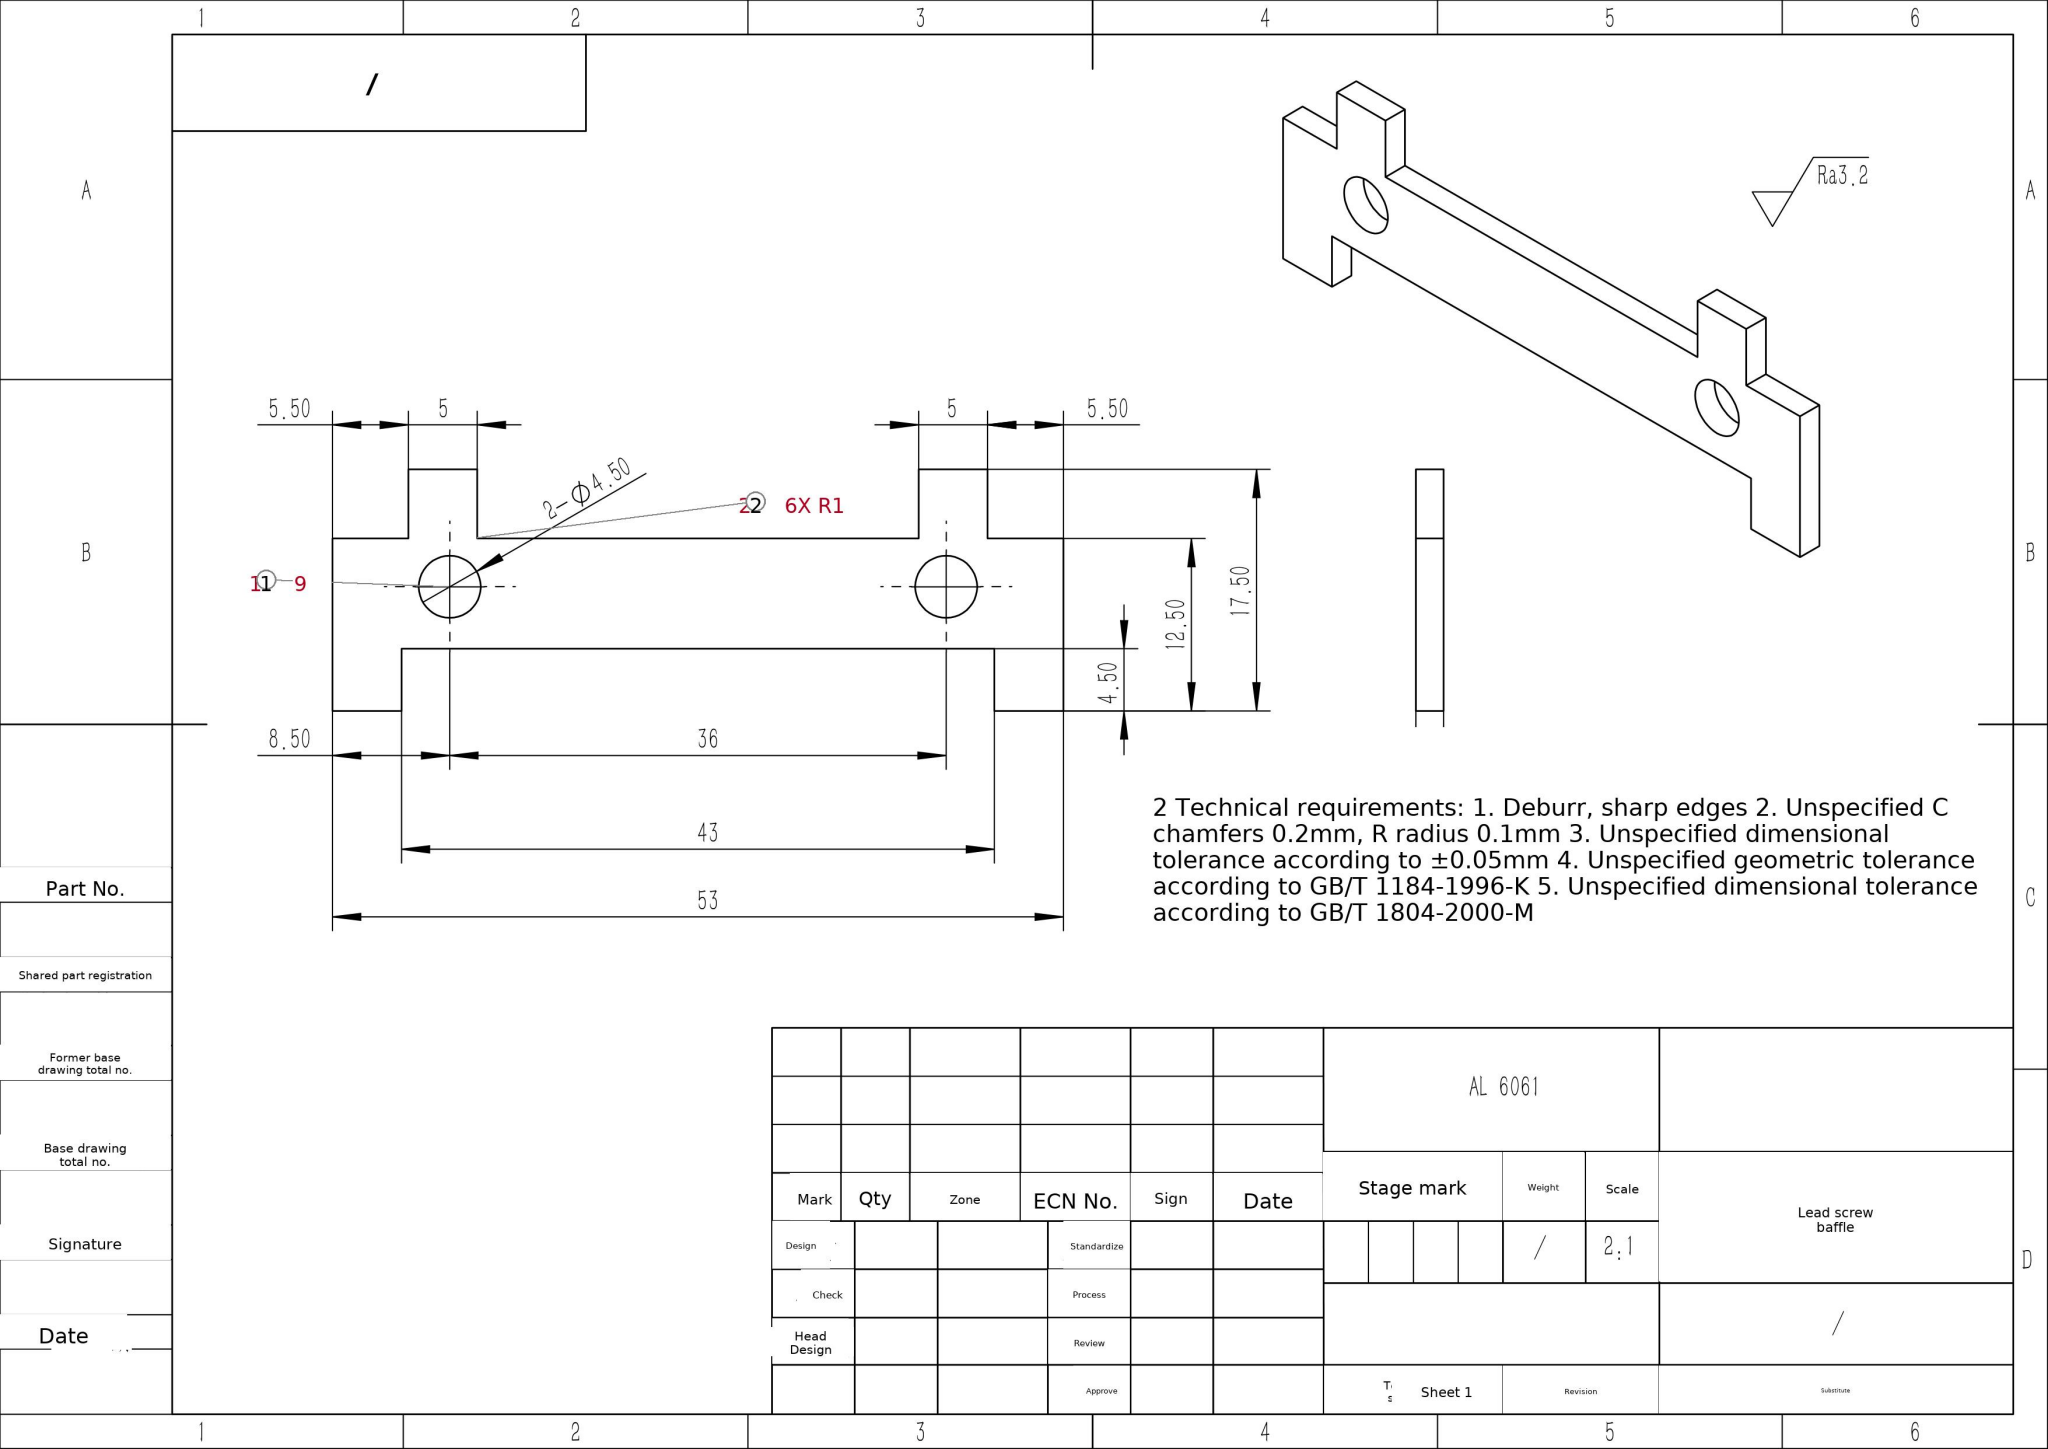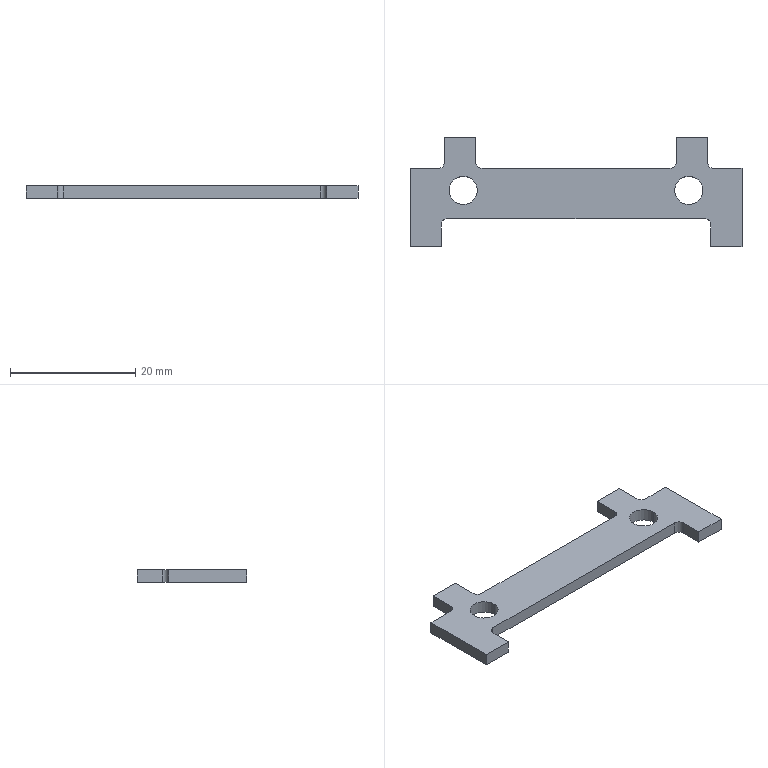Part | SolidWorks | mm | material AL 6061 | 1 solid | 28 faces | box 53 x 17.5 x 2 mm | volume 977 mm3 | plane 18 | cylinder 10 | commonest cylinder face diameters 2 x6 4.5 x4
build123d program:
from build123d import *

# Parameters (mm, degrees)
SKETCH1_R           = 2.25
BOSS_EXTRUDE1_DEPTH = 2
MOVE_FACE1_BY       = 0.5
MOVE_FACE1_2_BY     = 0.5
FILLET1_R           = 1


with BuildPart() as part:
    # Sketch1 → Boss-Extrude1 (new body)
    with BuildSketch(Plane.XY):
        Polygon((0, 0), (0, 13), (5.5, 13), (5.5, 18), (10.5, 18), (10.5, 13), (42.5, 13), (42.5, 18), (47.5, 18), (47.5, 13), (53, 13), (53, 0), (48, 0), (48, 5), (5, 5), (5, 0), align=None)
        with Locations((8.5, 9.496)):
            Circle(SKETCH1_R, mode=Mode.SUBTRACT)
        with Locations((44.5, 9.496)):
            Circle(SKETCH1_R, mode=Mode.SUBTRACT)
    extrude(amount=BOSS_EXTRUDE1_DEPTH)

    # Move Face1: a face moved inward by 0.5
    extrude(part.faces().sort_by_distance((2.5, 0, 1))[0], amount=MOVE_FACE1_BY, dir=(0, 1, 0), mode=Mode.SUBTRACT)

    # Move Face1 2: a face moved inward by 0.5
    extrude(part.faces().sort_by_distance((50.5, 0, 1))[0], amount=MOVE_FACE1_2_BY, dir=(0, 1, 0), mode=Mode.SUBTRACT)

    # Fillet1
    fillet1_edges = [part.edges().sort_by_distance(p)[0] for p in [
        (5.5, 13, 1),
        (10.5, 13, 1),
        (42.5, 13, 1),
        (47.5, 13, 1),
        (48, 5, 1),
        (5, 5, 1),
    ]]
    fillet(fillet1_edges, radius=FILLET1_R)


solid = part.part
STEP:
#1=CARTESIAN_POINT('',(42.25,9.496,2.));
#2=VERTEX_POINT('',#1);
#3=CARTESIAN_POINT('',(46.75,9.496,2.));
#4=VERTEX_POINT('',#3);
#5=CARTESIAN_POINT('',(44.5,9.496,2.));
#6=DIRECTION('',(0.,0.,1.));
#7=DIRECTION('',(1.,0.,0.));
#8=AXIS2_PLACEMENT_3D('',#5,#6,#7);
#9=CIRCLE('',#8,2.25);
#10=EDGE_CURVE('',#2,#4,#9,.T.);
#11=ORIENTED_EDGE('',*,*,#10,.T.);
#12=CARTESIAN_POINT('',(46.75,9.496,0.));
#13=VERTEX_POINT('',#12);
#14=CARTESIAN_POINT('',(46.75,9.496,2.));
#15=DIRECTION('',(0.,0.,-1.));
#16=VECTOR('',#15,1000.);
#17=LINE('',#14,#16);
#18=EDGE_CURVE('',#4,#13,#17,.T.);
#19=ORIENTED_EDGE('',*,*,#18,.T.);
#20=CARTESIAN_POINT('',(42.25,9.496,0.));
#21=VERTEX_POINT('',#20);
#22=CARTESIAN_POINT('',(44.5,9.496,0.));
#23=DIRECTION('',(0.,0.,1.));
#24=DIRECTION('',(1.,0.,0.));
#25=AXIS2_PLACEMENT_3D('',#22,#23,#24);
#26=CIRCLE('',#25,2.25);
#27=EDGE_CURVE('',#21,#13,#26,.T.);
#28=ORIENTED_EDGE('',*,*,#27,.F.);
#29=CARTESIAN_POINT('',(42.25,9.496,2.));
#30=DIRECTION('',(0.,0.,-1.));
#31=VECTOR('',#30,1000.);
#32=LINE('',#29,#31);
#33=EDGE_CURVE('',#2,#21,#32,.T.);
#34=ORIENTED_EDGE('',*,*,#33,.F.);
#35=EDGE_LOOP('',(#11,#19,#28,#34));
#36=FACE_OUTER_BOUND('',#35,.T.);
#37=CARTESIAN_POINT('',(44.5,9.496,2.));
#38=DIRECTION('',(0.,0.,-1.));
#39=DIRECTION('',(-1.,0.,0.));
#40=AXIS2_PLACEMENT_3D('',#37,#38,#39);
#41=CYLINDRICAL_SURFACE('',#40,2.25);
#42=ADVANCED_FACE('',(#36),#41,.F.);
#43=CARTESIAN_POINT('',(6.25,9.496,2.));
#44=VERTEX_POINT('',#43);
#45=CARTESIAN_POINT('',(10.75,9.496,2.));
#46=VERTEX_POINT('',#45);
#47=CARTESIAN_POINT('',(8.5,9.496,2.));
#48=DIRECTION('',(0.,0.,1.));
#49=DIRECTION('',(1.,0.,0.));
#50=AXIS2_PLACEMENT_3D('',#47,#48,#49);
#51=CIRCLE('',#50,2.25);
#52=EDGE_CURVE('',#44,#46,#51,.T.);
#53=ORIENTED_EDGE('',*,*,#52,.T.);
#54=CARTESIAN_POINT('',(10.75,9.496,0.));
#55=VERTEX_POINT('',#54);
#56=CARTESIAN_POINT('',(10.75,9.496,2.));
#57=DIRECTION('',(0.,0.,-1.));
#58=VECTOR('',#57,1000.);
#59=LINE('',#56,#58);
#60=EDGE_CURVE('',#46,#55,#59,.T.);
#61=ORIENTED_EDGE('',*,*,#60,.T.);
#62=CARTESIAN_POINT('',(6.25,9.496,0.));
#63=VERTEX_POINT('',#62);
#64=CARTESIAN_POINT('',(8.5,9.496,0.));
#65=DIRECTION('',(0.,0.,1.));
#66=DIRECTION('',(1.,0.,0.));
#67=AXIS2_PLACEMENT_3D('',#64,#65,#66);
#68=CIRCLE('',#67,2.25);
#69=EDGE_CURVE('',#63,#55,#68,.T.);
#70=ORIENTED_EDGE('',*,*,#69,.F.);
#71=CARTESIAN_POINT('',(6.25,9.496,2.));
#72=DIRECTION('',(0.,0.,-1.));
#73=VECTOR('',#72,1000.);
#74=LINE('',#71,#73);
#75=EDGE_CURVE('',#44,#63,#74,.T.);
#76=ORIENTED_EDGE('',*,*,#75,.F.);
#77=EDGE_LOOP('',(#53,#61,#70,#76));
#78=FACE_OUTER_BOUND('',#77,.T.);
#79=CARTESIAN_POINT('',(8.5,9.496,2.));
#80=DIRECTION('',(0.,0.,-1.));
#81=DIRECTION('',(-1.,0.,0.));
#82=AXIS2_PLACEMENT_3D('',#79,#80,#81);
#83=CYLINDRICAL_SURFACE('',#82,2.25);
#84=ADVANCED_FACE('',(#78),#83,.F.);
#85=CARTESIAN_POINT('',(0.,0.5,2.));
#86=VERTEX_POINT('',#85);
#87=CARTESIAN_POINT('',(5.,0.5,2.));
#88=VERTEX_POINT('',#87);
#89=CARTESIAN_POINT('',(5.,0.5,2.));
#90=DIRECTION('',(1.,-0.,0.));
#91=VECTOR('',#90,1000.);
#92=LINE('',#89,#91);
#93=EDGE_CURVE('',#86,#88,#92,.T.);
#94=ORIENTED_EDGE('',*,*,#93,.T.);
#95=CARTESIAN_POINT('',(5.,4.,2.));
#96=VERTEX_POINT('',#95);
#97=CARTESIAN_POINT('',(5.,5.,2.));
#98=DIRECTION('',(-0.,1.,0.));
#99=VECTOR('',#98,1000.);
#100=LINE('',#97,#99);
#101=EDGE_CURVE('',#88,#96,#100,.T.);
#102=ORIENTED_EDGE('',*,*,#101,.T.);
#103=CARTESIAN_POINT('',(6.,5.,2.));
#104=VERTEX_POINT('',#103);
#105=CARTESIAN_POINT('',(6.,4.,2.));
#106=DIRECTION('',(0.,0.,-1.));
#107=DIRECTION('',(-1.,0.,0.));
#108=AXIS2_PLACEMENT_3D('',#105,#106,#107);
#109=CIRCLE('',#108,1.);
#110=EDGE_CURVE('',#96,#104,#109,.T.);
#111=ORIENTED_EDGE('',*,*,#110,.T.);
#112=CARTESIAN_POINT('',(47.,5.,2.));
#113=VERTEX_POINT('',#112);
#114=CARTESIAN_POINT('',(48.,5.,2.));
#115=DIRECTION('',(1.,0.,0.));
#116=VECTOR('',#115,1000.);
#117=LINE('',#114,#116);
#118=EDGE_CURVE('',#104,#113,#117,.T.);
#119=ORIENTED_EDGE('',*,*,#118,.T.);
#120=CARTESIAN_POINT('',(48.,4.,2.));
#121=VERTEX_POINT('',#120);
#122=CARTESIAN_POINT('',(47.,4.,2.));
#123=DIRECTION('',(0.,0.,-1.));
#124=DIRECTION('',(-1.,0.,0.));
#125=AXIS2_PLACEMENT_3D('',#122,#123,#124);
#126=CIRCLE('',#125,1.);
#127=EDGE_CURVE('',#113,#121,#126,.T.);
#128=ORIENTED_EDGE('',*,*,#127,.T.);
#129=CARTESIAN_POINT('',(48.,0.5,2.));
#130=VERTEX_POINT('',#129);
#131=CARTESIAN_POINT('',(48.,-0.,2.));
#132=DIRECTION('',(0.,-1.,0.));
#133=VECTOR('',#132,1000.);
#134=LINE('',#131,#133);
#135=EDGE_CURVE('',#121,#130,#134,.T.);
#136=ORIENTED_EDGE('',*,*,#135,.T.);
#137=CARTESIAN_POINT('',(53.,0.5,2.));
#138=VERTEX_POINT('',#137);
#139=CARTESIAN_POINT('',(53.,0.5,2.));
#140=DIRECTION('',(1.,0.,0.));
#141=VECTOR('',#140,1000.);
#142=LINE('',#139,#141);
#143=EDGE_CURVE('',#130,#138,#142,.T.);
#144=ORIENTED_EDGE('',*,*,#143,.T.);
#145=CARTESIAN_POINT('',(53.,13.,2.));
#146=VERTEX_POINT('',#145);
#147=CARTESIAN_POINT('',(53.,13.,2.));
#148=DIRECTION('',(0.,1.,0.));
#149=VECTOR('',#148,1000.);
#150=LINE('',#147,#149);
#151=EDGE_CURVE('',#138,#146,#150,.T.);
#152=ORIENTED_EDGE('',*,*,#151,.T.);
#153=CARTESIAN_POINT('',(48.5,13.,2.));
#154=VERTEX_POINT('',#153);
#155=CARTESIAN_POINT('',(47.5,13.,2.));
#156=DIRECTION('',(-1.,0.,0.));
#157=VECTOR('',#156,1000.);
#158=LINE('',#155,#157);
#159=EDGE_CURVE('',#146,#154,#158,.T.);
#160=ORIENTED_EDGE('',*,*,#159,.T.);
#161=CARTESIAN_POINT('',(47.5,14.,2.));
#162=VERTEX_POINT('',#161);
#163=CARTESIAN_POINT('',(48.5,14.,2.));
#164=DIRECTION('',(0.,0.,-1.));
#165=DIRECTION('',(-1.,0.,0.));
#166=AXIS2_PLACEMENT_3D('',#163,#164,#165);
#167=CIRCLE('',#166,1.);
#168=EDGE_CURVE('',#154,#162,#167,.T.);
#169=ORIENTED_EDGE('',*,*,#168,.T.);
#170=CARTESIAN_POINT('',(47.5,18.,2.));
#171=VERTEX_POINT('',#170);
#172=CARTESIAN_POINT('',(47.5,18.,2.));
#173=DIRECTION('',(0.,1.,0.));
#174=VECTOR('',#173,1000.);
#175=LINE('',#172,#174);
#176=EDGE_CURVE('',#162,#171,#175,.T.);
#177=ORIENTED_EDGE('',*,*,#176,.T.);
#178=CARTESIAN_POINT('',(42.5,18.,2.));
#179=VERTEX_POINT('',#178);
#180=CARTESIAN_POINT('',(42.5,18.,2.));
#181=DIRECTION('',(-1.,-0.,0.));
#182=VECTOR('',#181,1000.);
#183=LINE('',#180,#182);
#184=EDGE_CURVE('',#171,#179,#183,.T.);
#185=ORIENTED_EDGE('',*,*,#184,.T.);
#186=CARTESIAN_POINT('',(42.5,14.,2.));
#187=VERTEX_POINT('',#186);
#188=CARTESIAN_POINT('',(42.5,13.,2.));
#189=DIRECTION('',(0.,-1.,0.));
#190=VECTOR('',#189,1000.);
#191=LINE('',#188,#190);
#192=EDGE_CURVE('',#179,#187,#191,.T.);
#193=ORIENTED_EDGE('',*,*,#192,.T.);
#194=CARTESIAN_POINT('',(41.5,13.,2.));
#195=VERTEX_POINT('',#194);
#196=CARTESIAN_POINT('',(41.5,14.,2.));
#197=DIRECTION('',(0.,0.,-1.));
#198=DIRECTION('',(-1.,0.,0.));
#199=AXIS2_PLACEMENT_3D('',#196,#197,#198);
#200=CIRCLE('',#199,1.);
#201=EDGE_CURVE('',#187,#195,#200,.T.);
#202=ORIENTED_EDGE('',*,*,#201,.T.);
#203=CARTESIAN_POINT('',(11.5,13.,2.));
#204=VERTEX_POINT('',#203);
#205=CARTESIAN_POINT('',(10.5,13.,2.));
#206=DIRECTION('',(-1.,0.,0.));
#207=VECTOR('',#206,1000.);
#208=LINE('',#205,#207);
#209=EDGE_CURVE('',#195,#204,#208,.T.);
#210=ORIENTED_EDGE('',*,*,#209,.T.);
#211=CARTESIAN_POINT('',(10.5,14.,2.));
#212=VERTEX_POINT('',#211);
#213=CARTESIAN_POINT('',(11.5,14.,2.));
#214=DIRECTION('',(0.,0.,-1.));
#215=DIRECTION('',(-1.,0.,0.));
#216=AXIS2_PLACEMENT_3D('',#213,#214,#215);
#217=CIRCLE('',#216,1.);
#218=EDGE_CURVE('',#204,#212,#217,.T.);
#219=ORIENTED_EDGE('',*,*,#218,.T.);
#220=CARTESIAN_POINT('',(10.5,18.,2.));
#221=VERTEX_POINT('',#220);
#222=CARTESIAN_POINT('',(10.5,18.,2.));
#223=DIRECTION('',(0.,1.,0.));
#224=VECTOR('',#223,1000.);
#225=LINE('',#222,#224);
#226=EDGE_CURVE('',#212,#221,#225,.T.);
#227=ORIENTED_EDGE('',*,*,#226,.T.);
#228=CARTESIAN_POINT('',(5.5,18.,2.));
#229=VERTEX_POINT('',#228);
#230=CARTESIAN_POINT('',(5.5,18.,2.));
#231=DIRECTION('',(-1.,0.,0.));
#232=VECTOR('',#231,1000.);
#233=LINE('',#230,#232);
#234=EDGE_CURVE('',#221,#229,#233,.T.);
#235=ORIENTED_EDGE('',*,*,#234,.T.);
#236=CARTESIAN_POINT('',(5.5,14.,2.));
#237=VERTEX_POINT('',#236);
#238=CARTESIAN_POINT('',(5.5,13.,2.));
#239=DIRECTION('',(0.,-1.,0.));
#240=VECTOR('',#239,1000.);
#241=LINE('',#238,#240);
#242=EDGE_CURVE('',#229,#237,#241,.T.);
#243=ORIENTED_EDGE('',*,*,#242,.T.);
#244=CARTESIAN_POINT('',(4.5,13.,2.));
#245=VERTEX_POINT('',#244);
#246=CARTESIAN_POINT('',(4.5,14.,2.));
#247=DIRECTION('',(0.,0.,-1.));
#248=DIRECTION('',(-1.,0.,0.));
#249=AXIS2_PLACEMENT_3D('',#246,#247,#248);
#250=CIRCLE('',#249,1.);
#251=EDGE_CURVE('',#237,#245,#250,.T.);
#252=ORIENTED_EDGE('',*,*,#251,.T.);
#253=CARTESIAN_POINT('',(0.,13.,2.));
#254=VERTEX_POINT('',#253);
#255=CARTESIAN_POINT('',(0.,13.,2.));
#256=DIRECTION('',(-1.,0.,0.));
#257=VECTOR('',#256,1000.);
#258=LINE('',#255,#257);
#259=EDGE_CURVE('',#245,#254,#258,.T.);
#260=ORIENTED_EDGE('',*,*,#259,.T.);
#261=CARTESIAN_POINT('',(0.,0.,2.));
#262=DIRECTION('',(0.,-1.,0.));
#263=VECTOR('',#262,1000.);
#264=LINE('',#261,#263);
#265=EDGE_CURVE('',#254,#86,#264,.T.);
#266=ORIENTED_EDGE('',*,*,#265,.T.);
#267=EDGE_LOOP('',(#94,#102,#111,#119,#128,#136,#144,#152,#160,#169,#177,#185,#193,#202,#210,#219,#227,#235,#243,#252,#260,#266));
#268=FACE_OUTER_BOUND('',#267,.T.);
#269=ORIENTED_EDGE('',*,*,#52,.F.);
#270=CARTESIAN_POINT('',(8.5,9.496,2.));
#271=DIRECTION('',(0.,0.,1.));
#272=DIRECTION('',(1.,0.,0.));
#273=AXIS2_PLACEMENT_3D('',#270,#271,#272);
#274=CIRCLE('',#273,2.25);
#275=EDGE_CURVE('',#46,#44,#274,.T.);
#276=ORIENTED_EDGE('',*,*,#275,.F.);
#277=EDGE_LOOP('',(#269,#276));
#278=FACE_BOUND('',#277,.T.);
#279=ORIENTED_EDGE('',*,*,#10,.F.);
#280=CARTESIAN_POINT('',(44.5,9.496,2.));
#281=DIRECTION('',(0.,0.,1.));
#282=DIRECTION('',(1.,0.,0.));
#283=AXIS2_PLACEMENT_3D('',#280,#281,#282);
#284=CIRCLE('',#283,2.25);
#285=EDGE_CURVE('',#4,#2,#284,.T.);
#286=ORIENTED_EDGE('',*,*,#285,.F.);
#287=EDGE_LOOP('',(#279,#286));
#288=FACE_BOUND('',#287,.T.);
#289=CARTESIAN_POINT('',(0.,0.,2.));
#290=DIRECTION('',(0.,0.,-1.));
#291=DIRECTION('',(-1.,0.,0.));
#292=AXIS2_PLACEMENT_3D('',#289,#290,#291);
#293=PLANE('',#292);
#294=ADVANCED_FACE('',(#268,#278,#288),#293,.F.);
#295=ORIENTED_EDGE('',*,*,#69,.T.);
#296=CARTESIAN_POINT('',(8.5,9.496,0.));
#297=DIRECTION('',(0.,0.,1.));
#298=DIRECTION('',(1.,0.,0.));
#299=AXIS2_PLACEMENT_3D('',#296,#297,#298);
#300=CIRCLE('',#299,2.25);
#301=EDGE_CURVE('',#55,#63,#300,.T.);
#302=ORIENTED_EDGE('',*,*,#301,.T.);
#303=EDGE_LOOP('',(#295,#302));
#304=FACE_BOUND('',#303,.T.);
#305=CARTESIAN_POINT('',(0.,0.5,0.));
#306=VERTEX_POINT('',#305);
#307=CARTESIAN_POINT('',(5.,0.5,0.));
#308=VERTEX_POINT('',#307);
#309=CARTESIAN_POINT('',(5.,0.5,0.));
#310=DIRECTION('',(1.,-0.,0.));
#311=VECTOR('',#310,1000.);
#312=LINE('',#309,#311);
#313=EDGE_CURVE('',#306,#308,#312,.T.);
#314=ORIENTED_EDGE('',*,*,#313,.F.);
#315=CARTESIAN_POINT('',(0.,13.,0.));
#316=VERTEX_POINT('',#315);
#317=CARTESIAN_POINT('',(0.,0.,0.));
#318=DIRECTION('',(0.,-1.,0.));
#319=VECTOR('',#318,1000.);
#320=LINE('',#317,#319);
#321=EDGE_CURVE('',#316,#306,#320,.T.);
#322=ORIENTED_EDGE('',*,*,#321,.F.);
#323=CARTESIAN_POINT('',(4.5,13.,0.));
#324=VERTEX_POINT('',#323);
#325=CARTESIAN_POINT('',(0.,13.,0.));
#326=DIRECTION('',(-1.,0.,0.));
#327=VECTOR('',#326,1000.);
#328=LINE('',#325,#327);
#329=EDGE_CURVE('',#324,#316,#328,.T.);
#330=ORIENTED_EDGE('',*,*,#329,.F.);
#331=CARTESIAN_POINT('',(5.5,14.,0.));
#332=VERTEX_POINT('',#331);
#333=CARTESIAN_POINT('',(4.5,14.,0.));
#334=DIRECTION('',(0.,0.,1.));
#335=DIRECTION('',(-1.,0.,0.));
#336=AXIS2_PLACEMENT_3D('',#333,#334,#335);
#337=CIRCLE('',#336,1.);
#338=EDGE_CURVE('',#324,#332,#337,.T.);
#339=ORIENTED_EDGE('',*,*,#338,.T.);
#340=CARTESIAN_POINT('',(5.5,18.,0.));
#341=VERTEX_POINT('',#340);
#342=CARTESIAN_POINT('',(5.5,13.,0.));
#343=DIRECTION('',(0.,-1.,0.));
#344=VECTOR('',#343,1000.);
#345=LINE('',#342,#344);
#346=EDGE_CURVE('',#341,#332,#345,.T.);
#347=ORIENTED_EDGE('',*,*,#346,.F.);
#348=CARTESIAN_POINT('',(10.5,18.,0.));
#349=VERTEX_POINT('',#348);
#350=CARTESIAN_POINT('',(5.5,18.,0.));
#351=DIRECTION('',(-1.,0.,0.));
#352=VECTOR('',#351,1000.);
#353=LINE('',#350,#352);
#354=EDGE_CURVE('',#349,#341,#353,.T.);
#355=ORIENTED_EDGE('',*,*,#354,.F.);
#356=CARTESIAN_POINT('',(10.5,14.,0.));
#357=VERTEX_POINT('',#356);
#358=CARTESIAN_POINT('',(10.5,18.,0.));
#359=DIRECTION('',(0.,1.,0.));
#360=VECTOR('',#359,1000.);
#361=LINE('',#358,#360);
#362=EDGE_CURVE('',#357,#349,#361,.T.);
#363=ORIENTED_EDGE('',*,*,#362,.F.);
#364=CARTESIAN_POINT('',(11.5,13.,0.));
#365=VERTEX_POINT('',#364);
#366=CARTESIAN_POINT('',(11.5,14.,0.));
#367=DIRECTION('',(0.,0.,1.));
#368=DIRECTION('',(-1.,0.,0.));
#369=AXIS2_PLACEMENT_3D('',#366,#367,#368);
#370=CIRCLE('',#369,1.);
#371=EDGE_CURVE('',#357,#365,#370,.T.);
#372=ORIENTED_EDGE('',*,*,#371,.T.);
#373=CARTESIAN_POINT('',(41.5,13.,0.));
#374=VERTEX_POINT('',#373);
#375=CARTESIAN_POINT('',(10.5,13.,0.));
#376=DIRECTION('',(-1.,0.,0.));
#377=VECTOR('',#376,1000.);
#378=LINE('',#375,#377);
#379=EDGE_CURVE('',#374,#365,#378,.T.);
#380=ORIENTED_EDGE('',*,*,#379,.F.);
#381=CARTESIAN_POINT('',(42.5,14.,0.));
#382=VERTEX_POINT('',#381);
#383=CARTESIAN_POINT('',(41.5,14.,0.));
#384=DIRECTION('',(0.,0.,1.));
#385=DIRECTION('',(-1.,0.,0.));
#386=AXIS2_PLACEMENT_3D('',#383,#384,#385);
#387=CIRCLE('',#386,1.);
#388=EDGE_CURVE('',#374,#382,#387,.T.);
#389=ORIENTED_EDGE('',*,*,#388,.T.);
#390=CARTESIAN_POINT('',(42.5,18.,0.));
#391=VERTEX_POINT('',#390);
#392=CARTESIAN_POINT('',(42.5,13.,0.));
#393=DIRECTION('',(0.,-1.,0.));
#394=VECTOR('',#393,1000.);
#395=LINE('',#392,#394);
#396=EDGE_CURVE('',#391,#382,#395,.T.);
#397=ORIENTED_EDGE('',*,*,#396,.F.);
#398=CARTESIAN_POINT('',(47.5,18.,0.));
#399=VERTEX_POINT('',#398);
#400=CARTESIAN_POINT('',(42.5,18.,0.));
#401=DIRECTION('',(-1.,-0.,0.));
#402=VECTOR('',#401,1000.);
#403=LINE('',#400,#402);
#404=EDGE_CURVE('',#399,#391,#403,.T.);
#405=ORIENTED_EDGE('',*,*,#404,.F.);
#406=CARTESIAN_POINT('',(47.5,14.,0.));
#407=VERTEX_POINT('',#406);
#408=CARTESIAN_POINT('',(47.5,18.,0.));
#409=DIRECTION('',(0.,1.,0.));
#410=VECTOR('',#409,1000.);
#411=LINE('',#408,#410);
#412=EDGE_CURVE('',#407,#399,#411,.T.);
#413=ORIENTED_EDGE('',*,*,#412,.F.);
#414=CARTESIAN_POINT('',(48.5,13.,0.));
#415=VERTEX_POINT('',#414);
#416=CARTESIAN_POINT('',(48.5,14.,0.));
#417=DIRECTION('',(0.,0.,1.));
#418=DIRECTION('',(-1.,0.,0.));
#419=AXIS2_PLACEMENT_3D('',#416,#417,#418);
#420=CIRCLE('',#419,1.);
#421=EDGE_CURVE('',#407,#415,#420,.T.);
#422=ORIENTED_EDGE('',*,*,#421,.T.);
#423=CARTESIAN_POINT('',(53.,13.,0.));
#424=VERTEX_POINT('',#423);
#425=CARTESIAN_POINT('',(47.5,13.,0.));
#426=DIRECTION('',(-1.,0.,0.));
#427=VECTOR('',#426,1000.);
#428=LINE('',#425,#427);
#429=EDGE_CURVE('',#424,#415,#428,.T.);
#430=ORIENTED_EDGE('',*,*,#429,.F.);
#431=CARTESIAN_POINT('',(53.,0.5,0.));
#432=VERTEX_POINT('',#431);
#433=CARTESIAN_POINT('',(53.,13.,0.));
#434=DIRECTION('',(0.,1.,0.));
#435=VECTOR('',#434,1000.);
#436=LINE('',#433,#435);
#437=EDGE_CURVE('',#432,#424,#436,.T.);
#438=ORIENTED_EDGE('',*,*,#437,.F.);
#439=CARTESIAN_POINT('',(48.,0.5,0.));
#440=VERTEX_POINT('',#439);
#441=CARTESIAN_POINT('',(53.,0.5,0.));
#442=DIRECTION('',(1.,0.,0.));
#443=VECTOR('',#442,1000.);
#444=LINE('',#441,#443);
#445=EDGE_CURVE('',#440,#432,#444,.T.);
#446=ORIENTED_EDGE('',*,*,#445,.F.);
#447=CARTESIAN_POINT('',(48.,4.,0.));
#448=VERTEX_POINT('',#447);
#449=CARTESIAN_POINT('',(48.,-0.,0.));
#450=DIRECTION('',(0.,-1.,0.));
#451=VECTOR('',#450,1000.);
#452=LINE('',#449,#451);
#453=EDGE_CURVE('',#448,#440,#452,.T.);
#454=ORIENTED_EDGE('',*,*,#453,.F.);
#455=CARTESIAN_POINT('',(47.,5.,0.));
#456=VERTEX_POINT('',#455);
#457=CARTESIAN_POINT('',(47.,4.,0.));
#458=DIRECTION('',(0.,0.,1.));
#459=DIRECTION('',(-1.,0.,0.));
#460=AXIS2_PLACEMENT_3D('',#457,#458,#459);
#461=CIRCLE('',#460,1.);
#462=EDGE_CURVE('',#448,#456,#461,.T.);
#463=ORIENTED_EDGE('',*,*,#462,.T.);
#464=CARTESIAN_POINT('',(6.,5.,0.));
#465=VERTEX_POINT('',#464);
#466=CARTESIAN_POINT('',(48.,5.,0.));
#467=DIRECTION('',(1.,0.,0.));
#468=VECTOR('',#467,1000.);
#469=LINE('',#466,#468);
#470=EDGE_CURVE('',#465,#456,#469,.T.);
#471=ORIENTED_EDGE('',*,*,#470,.F.);
#472=CARTESIAN_POINT('',(5.,4.,0.));
#473=VERTEX_POINT('',#472);
#474=CARTESIAN_POINT('',(6.,4.,0.));
#475=DIRECTION('',(0.,0.,1.));
#476=DIRECTION('',(-1.,-0.,0.));
#477=AXIS2_PLACEMENT_3D('',#474,#475,#476);
#478=CIRCLE('',#477,1.);
#479=EDGE_CURVE('',#465,#473,#478,.T.);
#480=ORIENTED_EDGE('',*,*,#479,.T.);
#481=CARTESIAN_POINT('',(5.,5.,0.));
#482=DIRECTION('',(-0.,1.,0.));
#483=VECTOR('',#482,1000.);
#484=LINE('',#481,#483);
#485=EDGE_CURVE('',#308,#473,#484,.T.);
#486=ORIENTED_EDGE('',*,*,#485,.F.);
#487=EDGE_LOOP('',(#314,#322,#330,#339,#347,#355,#363,#372,#380,#389,#397,#405,#413,#422,#430,#438,#446,#454,#463,#471,#480,#486));
#488=FACE_OUTER_BOUND('',#487,.T.);
#489=ORIENTED_EDGE('',*,*,#27,.T.);
#490=CARTESIAN_POINT('',(44.5,9.496,0.));
#491=DIRECTION('',(0.,0.,1.));
#492=DIRECTION('',(1.,0.,0.));
#493=AXIS2_PLACEMENT_3D('',#490,#491,#492);
#494=CIRCLE('',#493,2.25);
#495=EDGE_CURVE('',#13,#21,#494,.T.);
#496=ORIENTED_EDGE('',*,*,#495,.T.);
#497=EDGE_LOOP('',(#489,#496));
#498=FACE_BOUND('',#497,.T.);
#499=CARTESIAN_POINT('',(0.,0.,0.));
#500=DIRECTION('',(0.,0.,-1.));
#501=DIRECTION('',(-1.,0.,0.));
#502=AXIS2_PLACEMENT_3D('',#499,#500,#501);
#503=PLANE('',#502);
#504=ADVANCED_FACE('',(#304,#488,#498),#503,.T.);
#505=ORIENTED_EDGE('',*,*,#313,.T.);
#506=CARTESIAN_POINT('',(5.,0.5,2.));
#507=DIRECTION('',(0.,0.,-1.));
#508=VECTOR('',#507,1000.);
#509=LINE('',#506,#508);
#510=EDGE_CURVE('',#88,#308,#509,.T.);
#511=ORIENTED_EDGE('',*,*,#510,.F.);
#512=ORIENTED_EDGE('',*,*,#93,.F.);
#513=CARTESIAN_POINT('',(0.,0.5,2.));
#514=DIRECTION('',(0.,0.,-1.));
#515=VECTOR('',#514,1000.);
#516=LINE('',#513,#515);
#517=EDGE_CURVE('',#86,#306,#516,.T.);
#518=ORIENTED_EDGE('',*,*,#517,.T.);
#519=EDGE_LOOP('',(#505,#511,#512,#518));
#520=FACE_OUTER_BOUND('',#519,.T.);
#521=CARTESIAN_POINT('',(5.,0.5,2.));
#522=DIRECTION('',(0.,1.,0.));
#523=DIRECTION('',(-1.,0.,0.));
#524=AXIS2_PLACEMENT_3D('',#521,#522,#523);
#525=PLANE('',#524);
#526=ADVANCED_FACE('',(#520),#525,.F.);
#527=ORIENTED_EDGE('',*,*,#485,.T.);
#528=CARTESIAN_POINT('',(5.,4.,2.));
#529=DIRECTION('',(0.,0.,1.));
#530=VECTOR('',#529,1000.);
#531=LINE('',#528,#530);
#532=EDGE_CURVE('',#473,#96,#531,.T.);
#533=ORIENTED_EDGE('',*,*,#532,.T.);
#534=ORIENTED_EDGE('',*,*,#101,.F.);
#535=ORIENTED_EDGE('',*,*,#510,.T.);
#536=EDGE_LOOP('',(#527,#533,#534,#535));
#537=FACE_OUTER_BOUND('',#536,.T.);
#538=CARTESIAN_POINT('',(5.,5.,2.));
#539=DIRECTION('',(-1.,-0.,0.));
#540=DIRECTION('',(0.,-1.,0.));
#541=AXIS2_PLACEMENT_3D('',#538,#539,#540);
#542=PLANE('',#541);
#543=ADVANCED_FACE('',(#537),#542,.F.);
#544=ORIENTED_EDGE('',*,*,#118,.F.);
#545=CARTESIAN_POINT('',(6.,5.,0.));
#546=DIRECTION('',(0.,0.,-1.));
#547=VECTOR('',#546,1000.);
#548=LINE('',#545,#547);
#549=EDGE_CURVE('',#104,#465,#548,.T.);
#550=ORIENTED_EDGE('',*,*,#549,.T.);
#551=ORIENTED_EDGE('',*,*,#470,.T.);
#552=CARTESIAN_POINT('',(47.,5.,2.));
#553=DIRECTION('',(0.,0.,1.));
#554=VECTOR('',#553,1000.);
#555=LINE('',#552,#554);
#556=EDGE_CURVE('',#456,#113,#555,.T.);
#557=ORIENTED_EDGE('',*,*,#556,.T.);
#558=EDGE_LOOP('',(#544,#550,#551,#557));
#559=FACE_OUTER_BOUND('',#558,.T.);
#560=CARTESIAN_POINT('',(48.,5.,2.));
#561=DIRECTION('',(-0.,1.,0.));
#562=DIRECTION('',(-1.,-0.,0.));
#563=AXIS2_PLACEMENT_3D('',#560,#561,#562);
#564=PLANE('',#563);
#565=ADVANCED_FACE('',(#559),#564,.F.);
#566=ORIENTED_EDGE('',*,*,#135,.F.);
#567=CARTESIAN_POINT('',(48.,4.,0.));
#568=DIRECTION('',(0.,0.,-1.));
#569=VECTOR('',#568,1000.);
#570=LINE('',#567,#569);
#571=EDGE_CURVE('',#121,#448,#570,.T.);
#572=ORIENTED_EDGE('',*,*,#571,.T.);
#573=ORIENTED_EDGE('',*,*,#453,.T.);
#574=CARTESIAN_POINT('',(48.,0.5,2.));
#575=DIRECTION('',(0.,0.,-1.));
#576=VECTOR('',#575,1000.);
#577=LINE('',#574,#576);
#578=EDGE_CURVE('',#130,#440,#577,.T.);
#579=ORIENTED_EDGE('',*,*,#578,.F.);
#580=EDGE_LOOP('',(#566,#572,#573,#579));
#581=FACE_OUTER_BOUND('',#580,.T.);
#582=CARTESIAN_POINT('',(48.,-0.,2.));
#583=DIRECTION('',(1.,0.,0.));
#584=DIRECTION('',(0.,0.,-1.));
#585=AXIS2_PLACEMENT_3D('',#582,#583,#584);
#586=PLANE('',#585);
#587=ADVANCED_FACE('',(#581),#586,.F.);
#588=ORIENTED_EDGE('',*,*,#445,.T.);
#589=CARTESIAN_POINT('',(53.,0.5,2.));
#590=DIRECTION('',(0.,0.,-1.));
#591=VECTOR('',#590,1000.);
#592=LINE('',#589,#591);
#593=EDGE_CURVE('',#138,#432,#592,.T.);
#594=ORIENTED_EDGE('',*,*,#593,.F.);
#595=ORIENTED_EDGE('',*,*,#143,.F.);
#596=ORIENTED_EDGE('',*,*,#578,.T.);
#597=EDGE_LOOP('',(#588,#594,#595,#596));
#598=FACE_OUTER_BOUND('',#597,.T.);
#599=CARTESIAN_POINT('',(53.,0.5,2.));
#600=DIRECTION('',(-0.,1.,0.));
#601=DIRECTION('',(-1.,-0.,0.));
#602=AXIS2_PLACEMENT_3D('',#599,#600,#601);
#603=PLANE('',#602);
#604=ADVANCED_FACE('',(#598),#603,.F.);
#605=ORIENTED_EDGE('',*,*,#437,.T.);
#606=CARTESIAN_POINT('',(53.,13.,2.));
#607=DIRECTION('',(0.,0.,-1.));
#608=VECTOR('',#607,1000.);
#609=LINE('',#606,#608);
#610=EDGE_CURVE('',#146,#424,#609,.T.);
#611=ORIENTED_EDGE('',*,*,#610,.F.);
#612=ORIENTED_EDGE('',*,*,#151,.F.);
#613=ORIENTED_EDGE('',*,*,#593,.T.);
#614=EDGE_LOOP('',(#605,#611,#612,#613));
#615=FACE_OUTER_BOUND('',#614,.T.);
#616=CARTESIAN_POINT('',(53.,13.,2.));
#617=DIRECTION('',(-1.,0.,0.));
#618=DIRECTION('',(0.,0.,1.));
#619=AXIS2_PLACEMENT_3D('',#616,#617,#618);
#620=PLANE('',#619);
#621=ADVANCED_FACE('',(#615),#620,.F.);
#622=ORIENTED_EDGE('',*,*,#429,.T.);
#623=CARTESIAN_POINT('',(48.5,13.,2.));
#624=DIRECTION('',(0.,0.,1.));
#625=VECTOR('',#624,1000.);
#626=LINE('',#623,#625);
#627=EDGE_CURVE('',#415,#154,#626,.T.);
#628=ORIENTED_EDGE('',*,*,#627,.T.);
#629=ORIENTED_EDGE('',*,*,#159,.F.);
#630=ORIENTED_EDGE('',*,*,#610,.T.);
#631=EDGE_LOOP('',(#622,#628,#629,#630));
#632=FACE_OUTER_BOUND('',#631,.T.);
#633=CARTESIAN_POINT('',(47.5,13.,2.));
#634=DIRECTION('',(0.,-1.,0.));
#635=DIRECTION('',(0.,0.,-1.));
#636=AXIS2_PLACEMENT_3D('',#633,#634,#635);
#637=PLANE('',#636);
#638=ADVANCED_FACE('',(#632),#637,.F.);
#639=ORIENTED_EDGE('',*,*,#176,.F.);
#640=CARTESIAN_POINT('',(47.5,14.,0.));
#641=DIRECTION('',(0.,0.,-1.));
#642=VECTOR('',#641,1000.);
#643=LINE('',#640,#642);
#644=EDGE_CURVE('',#162,#407,#643,.T.);
#645=ORIENTED_EDGE('',*,*,#644,.T.);
#646=ORIENTED_EDGE('',*,*,#412,.T.);
#647=CARTESIAN_POINT('',(47.5,18.,2.));
#648=DIRECTION('',(0.,0.,-1.));
#649=VECTOR('',#648,1000.);
#650=LINE('',#647,#649);
#651=EDGE_CURVE('',#171,#399,#650,.T.);
#652=ORIENTED_EDGE('',*,*,#651,.F.);
#653=EDGE_LOOP('',(#639,#645,#646,#652));
#654=FACE_OUTER_BOUND('',#653,.T.);
#655=CARTESIAN_POINT('',(47.5,18.,2.));
#656=DIRECTION('',(-1.,0.,0.));
#657=DIRECTION('',(0.,0.,1.));
#658=AXIS2_PLACEMENT_3D('',#655,#656,#657);
#659=PLANE('',#658);
#660=ADVANCED_FACE('',(#654),#659,.F.);
#661=ORIENTED_EDGE('',*,*,#404,.T.);
#662=CARTESIAN_POINT('',(42.5,18.,2.));
#663=DIRECTION('',(0.,0.,-1.));
#664=VECTOR('',#663,1000.);
#665=LINE('',#662,#664);
#666=EDGE_CURVE('',#179,#391,#665,.T.);
#667=ORIENTED_EDGE('',*,*,#666,.F.);
#668=ORIENTED_EDGE('',*,*,#184,.F.);
#669=ORIENTED_EDGE('',*,*,#651,.T.);
#670=EDGE_LOOP('',(#661,#667,#668,#669));
#671=FACE_OUTER_BOUND('',#670,.T.);
#672=CARTESIAN_POINT('',(42.5,18.,2.));
#673=DIRECTION('',(0.,-1.,0.));
#674=DIRECTION('',(1.,0.,0.));
#675=AXIS2_PLACEMENT_3D('',#672,#673,#674);
#676=PLANE('',#675);
#677=ADVANCED_FACE('',(#671),#676,.F.);
#678=ORIENTED_EDGE('',*,*,#396,.T.);
#679=CARTESIAN_POINT('',(42.5,14.,2.));
#680=DIRECTION('',(0.,0.,1.));
#681=VECTOR('',#680,1000.);
#682=LINE('',#679,#681);
#683=EDGE_CURVE('',#382,#187,#682,.T.);
#684=ORIENTED_EDGE('',*,*,#683,.T.);
#685=ORIENTED_EDGE('',*,*,#192,.F.);
#686=ORIENTED_EDGE('',*,*,#666,.T.);
#687=EDGE_LOOP('',(#678,#684,#685,#686));
#688=FACE_OUTER_BOUND('',#687,.T.);
#689=CARTESIAN_POINT('',(42.5,13.,2.));
#690=DIRECTION('',(1.,0.,0.));
#691=DIRECTION('',(0.,0.,-1.));
#692=AXIS2_PLACEMENT_3D('',#689,#690,#691);
#693=PLANE('',#692);
#694=ADVANCED_FACE('',(#688),#693,.F.);
#695=ORIENTED_EDGE('',*,*,#209,.F.);
#696=CARTESIAN_POINT('',(41.5,13.,0.));
#697=DIRECTION('',(0.,0.,-1.));
#698=VECTOR('',#697,1000.);
#699=LINE('',#696,#698);
#700=EDGE_CURVE('',#195,#374,#699,.T.);
#701=ORIENTED_EDGE('',*,*,#700,.T.);
#702=ORIENTED_EDGE('',*,*,#379,.T.);
#703=CARTESIAN_POINT('',(11.5,13.,2.));
#704=DIRECTION('',(0.,0.,1.));
#705=VECTOR('',#704,1000.);
#706=LINE('',#703,#705);
#707=EDGE_CURVE('',#365,#204,#706,.T.);
#708=ORIENTED_EDGE('',*,*,#707,.T.);
#709=EDGE_LOOP('',(#695,#701,#702,#708));
#710=FACE_OUTER_BOUND('',#709,.T.);
#711=CARTESIAN_POINT('',(10.5,13.,2.));
#712=DIRECTION('',(0.,-1.,0.));
#713=DIRECTION('',(0.,0.,-1.));
#714=AXIS2_PLACEMENT_3D('',#711,#712,#713);
#715=PLANE('',#714);
#716=ADVANCED_FACE('',(#710),#715,.F.);
#717=ORIENTED_EDGE('',*,*,#226,.F.);
#718=CARTESIAN_POINT('',(10.5,14.,0.));
#719=DIRECTION('',(0.,0.,-1.));
#720=VECTOR('',#719,1000.);
#721=LINE('',#718,#720);
#722=EDGE_CURVE('',#212,#357,#721,.T.);
#723=ORIENTED_EDGE('',*,*,#722,.T.);
#724=ORIENTED_EDGE('',*,*,#362,.T.);
#725=CARTESIAN_POINT('',(10.5,18.,2.));
#726=DIRECTION('',(0.,0.,-1.));
#727=VECTOR('',#726,1000.);
#728=LINE('',#725,#727);
#729=EDGE_CURVE('',#221,#349,#728,.T.);
#730=ORIENTED_EDGE('',*,*,#729,.F.);
#731=EDGE_LOOP('',(#717,#723,#724,#730));
#732=FACE_OUTER_BOUND('',#731,.T.);
#733=CARTESIAN_POINT('',(10.5,18.,2.));
#734=DIRECTION('',(-1.,0.,0.));
#735=DIRECTION('',(0.,0.,1.));
#736=AXIS2_PLACEMENT_3D('',#733,#734,#735);
#737=PLANE('',#736);
#738=ADVANCED_FACE('',(#732),#737,.F.);
#739=ORIENTED_EDGE('',*,*,#354,.T.);
#740=CARTESIAN_POINT('',(5.5,18.,2.));
#741=DIRECTION('',(0.,0.,-1.));
#742=VECTOR('',#741,1000.);
#743=LINE('',#740,#742);
#744=EDGE_CURVE('',#229,#341,#743,.T.);
#745=ORIENTED_EDGE('',*,*,#744,.F.);
#746=ORIENTED_EDGE('',*,*,#234,.F.);
#747=ORIENTED_EDGE('',*,*,#729,.T.);
#748=EDGE_LOOP('',(#739,#745,#746,#747));
#749=FACE_OUTER_BOUND('',#748,.T.);
#750=CARTESIAN_POINT('',(5.5,18.,2.));
#751=DIRECTION('',(0.,-1.,0.));
#752=DIRECTION('',(0.,0.,-1.));
#753=AXIS2_PLACEMENT_3D('',#750,#751,#752);
#754=PLANE('',#753);
#755=ADVANCED_FACE('',(#749),#754,.F.);
#756=ORIENTED_EDGE('',*,*,#346,.T.);
#757=CARTESIAN_POINT('',(5.5,14.,2.));
#758=DIRECTION('',(0.,0.,1.));
#759=VECTOR('',#758,1000.);
#760=LINE('',#757,#759);
#761=EDGE_CURVE('',#332,#237,#760,.T.);
#762=ORIENTED_EDGE('',*,*,#761,.T.);
#763=ORIENTED_EDGE('',*,*,#242,.F.);
#764=ORIENTED_EDGE('',*,*,#744,.T.);
#765=EDGE_LOOP('',(#756,#762,#763,#764));
#766=FACE_OUTER_BOUND('',#765,.T.);
#767=CARTESIAN_POINT('',(5.5,13.,2.));
#768=DIRECTION('',(1.,0.,0.));
#769=DIRECTION('',(0.,0.,-1.));
#770=AXIS2_PLACEMENT_3D('',#767,#768,#769);
#771=PLANE('',#770);
#772=ADVANCED_FACE('',(#766),#771,.F.);
#773=ORIENTED_EDGE('',*,*,#259,.F.);
#774=CARTESIAN_POINT('',(4.5,13.,0.));
#775=DIRECTION('',(0.,0.,-1.));
#776=VECTOR('',#775,1000.);
#777=LINE('',#774,#776);
#778=EDGE_CURVE('',#245,#324,#777,.T.);
#779=ORIENTED_EDGE('',*,*,#778,.T.);
#780=ORIENTED_EDGE('',*,*,#329,.T.);
#781=CARTESIAN_POINT('',(0.,13.,2.));
#782=DIRECTION('',(0.,0.,-1.));
#783=VECTOR('',#782,1000.);
#784=LINE('',#781,#783);
#785=EDGE_CURVE('',#254,#316,#784,.T.);
#786=ORIENTED_EDGE('',*,*,#785,.F.);
#787=EDGE_LOOP('',(#773,#779,#780,#786));
#788=FACE_OUTER_BOUND('',#787,.T.);
#789=CARTESIAN_POINT('',(0.,13.,2.));
#790=DIRECTION('',(0.,-1.,0.));
#791=DIRECTION('',(0.,0.,-1.));
#792=AXIS2_PLACEMENT_3D('',#789,#790,#791);
#793=PLANE('',#792);
#794=ADVANCED_FACE('',(#788),#793,.F.);
#795=ORIENTED_EDGE('',*,*,#321,.T.);
#796=ORIENTED_EDGE('',*,*,#517,.F.);
#797=ORIENTED_EDGE('',*,*,#265,.F.);
#798=ORIENTED_EDGE('',*,*,#785,.T.);
#799=EDGE_LOOP('',(#795,#796,#797,#798));
#800=FACE_OUTER_BOUND('',#799,.T.);
#801=CARTESIAN_POINT('',(0.,0.,2.));
#802=DIRECTION('',(1.,0.,0.));
#803=DIRECTION('',(0.,0.,-1.));
#804=AXIS2_PLACEMENT_3D('',#801,#802,#803);
#805=PLANE('',#804);
#806=ADVANCED_FACE('',(#800),#805,.F.);
#807=ORIENTED_EDGE('',*,*,#60,.F.);
#808=ORIENTED_EDGE('',*,*,#275,.T.);
#809=ORIENTED_EDGE('',*,*,#75,.T.);
#810=ORIENTED_EDGE('',*,*,#301,.F.);
#811=EDGE_LOOP('',(#807,#808,#809,#810));
#812=FACE_OUTER_BOUND('',#811,.T.);
#813=CARTESIAN_POINT('',(8.5,9.496,2.));
#814=DIRECTION('',(0.,0.,-1.));
#815=DIRECTION('',(-1.,0.,0.));
#816=AXIS2_PLACEMENT_3D('',#813,#814,#815);
#817=CYLINDRICAL_SURFACE('',#816,2.25);
#818=ADVANCED_FACE('',(#812),#817,.F.);
#819=ORIENTED_EDGE('',*,*,#18,.F.);
#820=ORIENTED_EDGE('',*,*,#285,.T.);
#821=ORIENTED_EDGE('',*,*,#33,.T.);
#822=ORIENTED_EDGE('',*,*,#495,.F.);
#823=EDGE_LOOP('',(#819,#820,#821,#822));
#824=FACE_OUTER_BOUND('',#823,.T.);
#825=CARTESIAN_POINT('',(44.5,9.496,2.));
#826=DIRECTION('',(0.,0.,-1.));
#827=DIRECTION('',(-1.,0.,0.));
#828=AXIS2_PLACEMENT_3D('',#825,#826,#827);
#829=CYLINDRICAL_SURFACE('',#828,2.25);
#830=ADVANCED_FACE('',(#824),#829,.F.);
#831=ORIENTED_EDGE('',*,*,#110,.F.);
#832=ORIENTED_EDGE('',*,*,#532,.F.);
#833=ORIENTED_EDGE('',*,*,#479,.F.);
#834=ORIENTED_EDGE('',*,*,#549,.F.);
#835=EDGE_LOOP('',(#831,#832,#833,#834));
#836=FACE_OUTER_BOUND('',#835,.T.);
#837=CARTESIAN_POINT('',(6.,4.,2.));
#838=DIRECTION('',(0.,0.,1.));
#839=DIRECTION('',(1.,0.,0.));
#840=AXIS2_PLACEMENT_3D('',#837,#838,#839);
#841=CYLINDRICAL_SURFACE('',#840,1.);
#842=ADVANCED_FACE('',(#836),#841,.F.);
#843=ORIENTED_EDGE('',*,*,#127,.F.);
#844=ORIENTED_EDGE('',*,*,#556,.F.);
#845=ORIENTED_EDGE('',*,*,#462,.F.);
#846=ORIENTED_EDGE('',*,*,#571,.F.);
#847=EDGE_LOOP('',(#843,#844,#845,#846));
#848=FACE_OUTER_BOUND('',#847,.T.);
#849=CARTESIAN_POINT('',(47.,4.,2.));
#850=DIRECTION('',(0.,0.,1.));
#851=DIRECTION('',(1.,0.,0.));
#852=AXIS2_PLACEMENT_3D('',#849,#850,#851);
#853=CYLINDRICAL_SURFACE('',#852,1.);
#854=ADVANCED_FACE('',(#848),#853,.F.);
#855=ORIENTED_EDGE('',*,*,#201,.F.);
#856=ORIENTED_EDGE('',*,*,#683,.F.);
#857=ORIENTED_EDGE('',*,*,#388,.F.);
#858=ORIENTED_EDGE('',*,*,#700,.F.);
#859=EDGE_LOOP('',(#855,#856,#857,#858));
#860=FACE_OUTER_BOUND('',#859,.T.);
#861=CARTESIAN_POINT('',(41.5,14.,2.));
#862=DIRECTION('',(0.,0.,1.));
#863=DIRECTION('',(1.,0.,0.));
#864=AXIS2_PLACEMENT_3D('',#861,#862,#863);
#865=CYLINDRICAL_SURFACE('',#864,1.);
#866=ADVANCED_FACE('',(#860),#865,.F.);
#867=ORIENTED_EDGE('',*,*,#168,.F.);
#868=ORIENTED_EDGE('',*,*,#627,.F.);
#869=ORIENTED_EDGE('',*,*,#421,.F.);
#870=ORIENTED_EDGE('',*,*,#644,.F.);
#871=EDGE_LOOP('',(#867,#868,#869,#870));
#872=FACE_OUTER_BOUND('',#871,.T.);
#873=CARTESIAN_POINT('',(48.5,14.,2.));
#874=DIRECTION('',(0.,0.,1.));
#875=DIRECTION('',(1.,0.,0.));
#876=AXIS2_PLACEMENT_3D('',#873,#874,#875);
#877=CYLINDRICAL_SURFACE('',#876,1.);
#878=ADVANCED_FACE('',(#872),#877,.F.);
#879=ORIENTED_EDGE('',*,*,#218,.F.);
#880=ORIENTED_EDGE('',*,*,#707,.F.);
#881=ORIENTED_EDGE('',*,*,#371,.F.);
#882=ORIENTED_EDGE('',*,*,#722,.F.);
#883=EDGE_LOOP('',(#879,#880,#881,#882));
#884=FACE_OUTER_BOUND('',#883,.T.);
#885=CARTESIAN_POINT('',(11.5,14.,2.));
#886=DIRECTION('',(0.,0.,1.));
#887=DIRECTION('',(1.,0.,0.));
#888=AXIS2_PLACEMENT_3D('',#885,#886,#887);
#889=CYLINDRICAL_SURFACE('',#888,1.);
#890=ADVANCED_FACE('',(#884),#889,.F.);
#891=ORIENTED_EDGE('',*,*,#251,.F.);
#892=ORIENTED_EDGE('',*,*,#761,.F.);
#893=ORIENTED_EDGE('',*,*,#338,.F.);
#894=ORIENTED_EDGE('',*,*,#778,.F.);
#895=EDGE_LOOP('',(#891,#892,#893,#894));
#896=FACE_OUTER_BOUND('',#895,.T.);
#897=CARTESIAN_POINT('',(4.5,14.,2.));
#898=DIRECTION('',(0.,0.,1.));
#899=DIRECTION('',(1.,0.,0.));
#900=AXIS2_PLACEMENT_3D('',#897,#898,#899);
#901=CYLINDRICAL_SURFACE('',#900,1.);
#902=ADVANCED_FACE('',(#896),#901,.F.);
#903=CLOSED_SHELL('',(#42,#84,#294,#504,#526,#543,#565,#587,#604,#621,#638,#660,#677,#694,#716,#738,#755,#772,#794,#806,#818,#830,#842,#854,#866,#878,#890,#902));
#904=MANIFOLD_SOLID_BREP('',#903);
#905=CARTESIAN_POINT('',(0.,0.,0.));
#906=DIRECTION('',(0.,0.,1.));
#907=DIRECTION('',(1.,0.,0.));
#908=AXIS2_PLACEMENT_3D('',#905,#906,#907);
#909=(LENGTH_UNIT()NAMED_UNIT(*)SI_UNIT(.MILLI.,.METRE.));
#910=UNCERTAINTY_MEASURE_WITH_UNIT(LENGTH_MEASURE(0.00001),#909,'','');
#911=(NAMED_UNIT(*)PLANE_ANGLE_UNIT()SI_UNIT($,.RADIAN.));
#912=(NAMED_UNIT(*)SI_UNIT($,.STERADIAN.)SOLID_ANGLE_UNIT());
#913=(GEOMETRIC_REPRESENTATION_CONTEXT(3)GLOBAL_UNCERTAINTY_ASSIGNED_CONTEXT((#910))GLOBAL_UNIT_ASSIGNED_CONTEXT((#909,#911,#912))REPRESENTATION_CONTEXT('',''));
#914=ADVANCED_BREP_SHAPE_REPRESENTATION('',(#904,#908),#913);